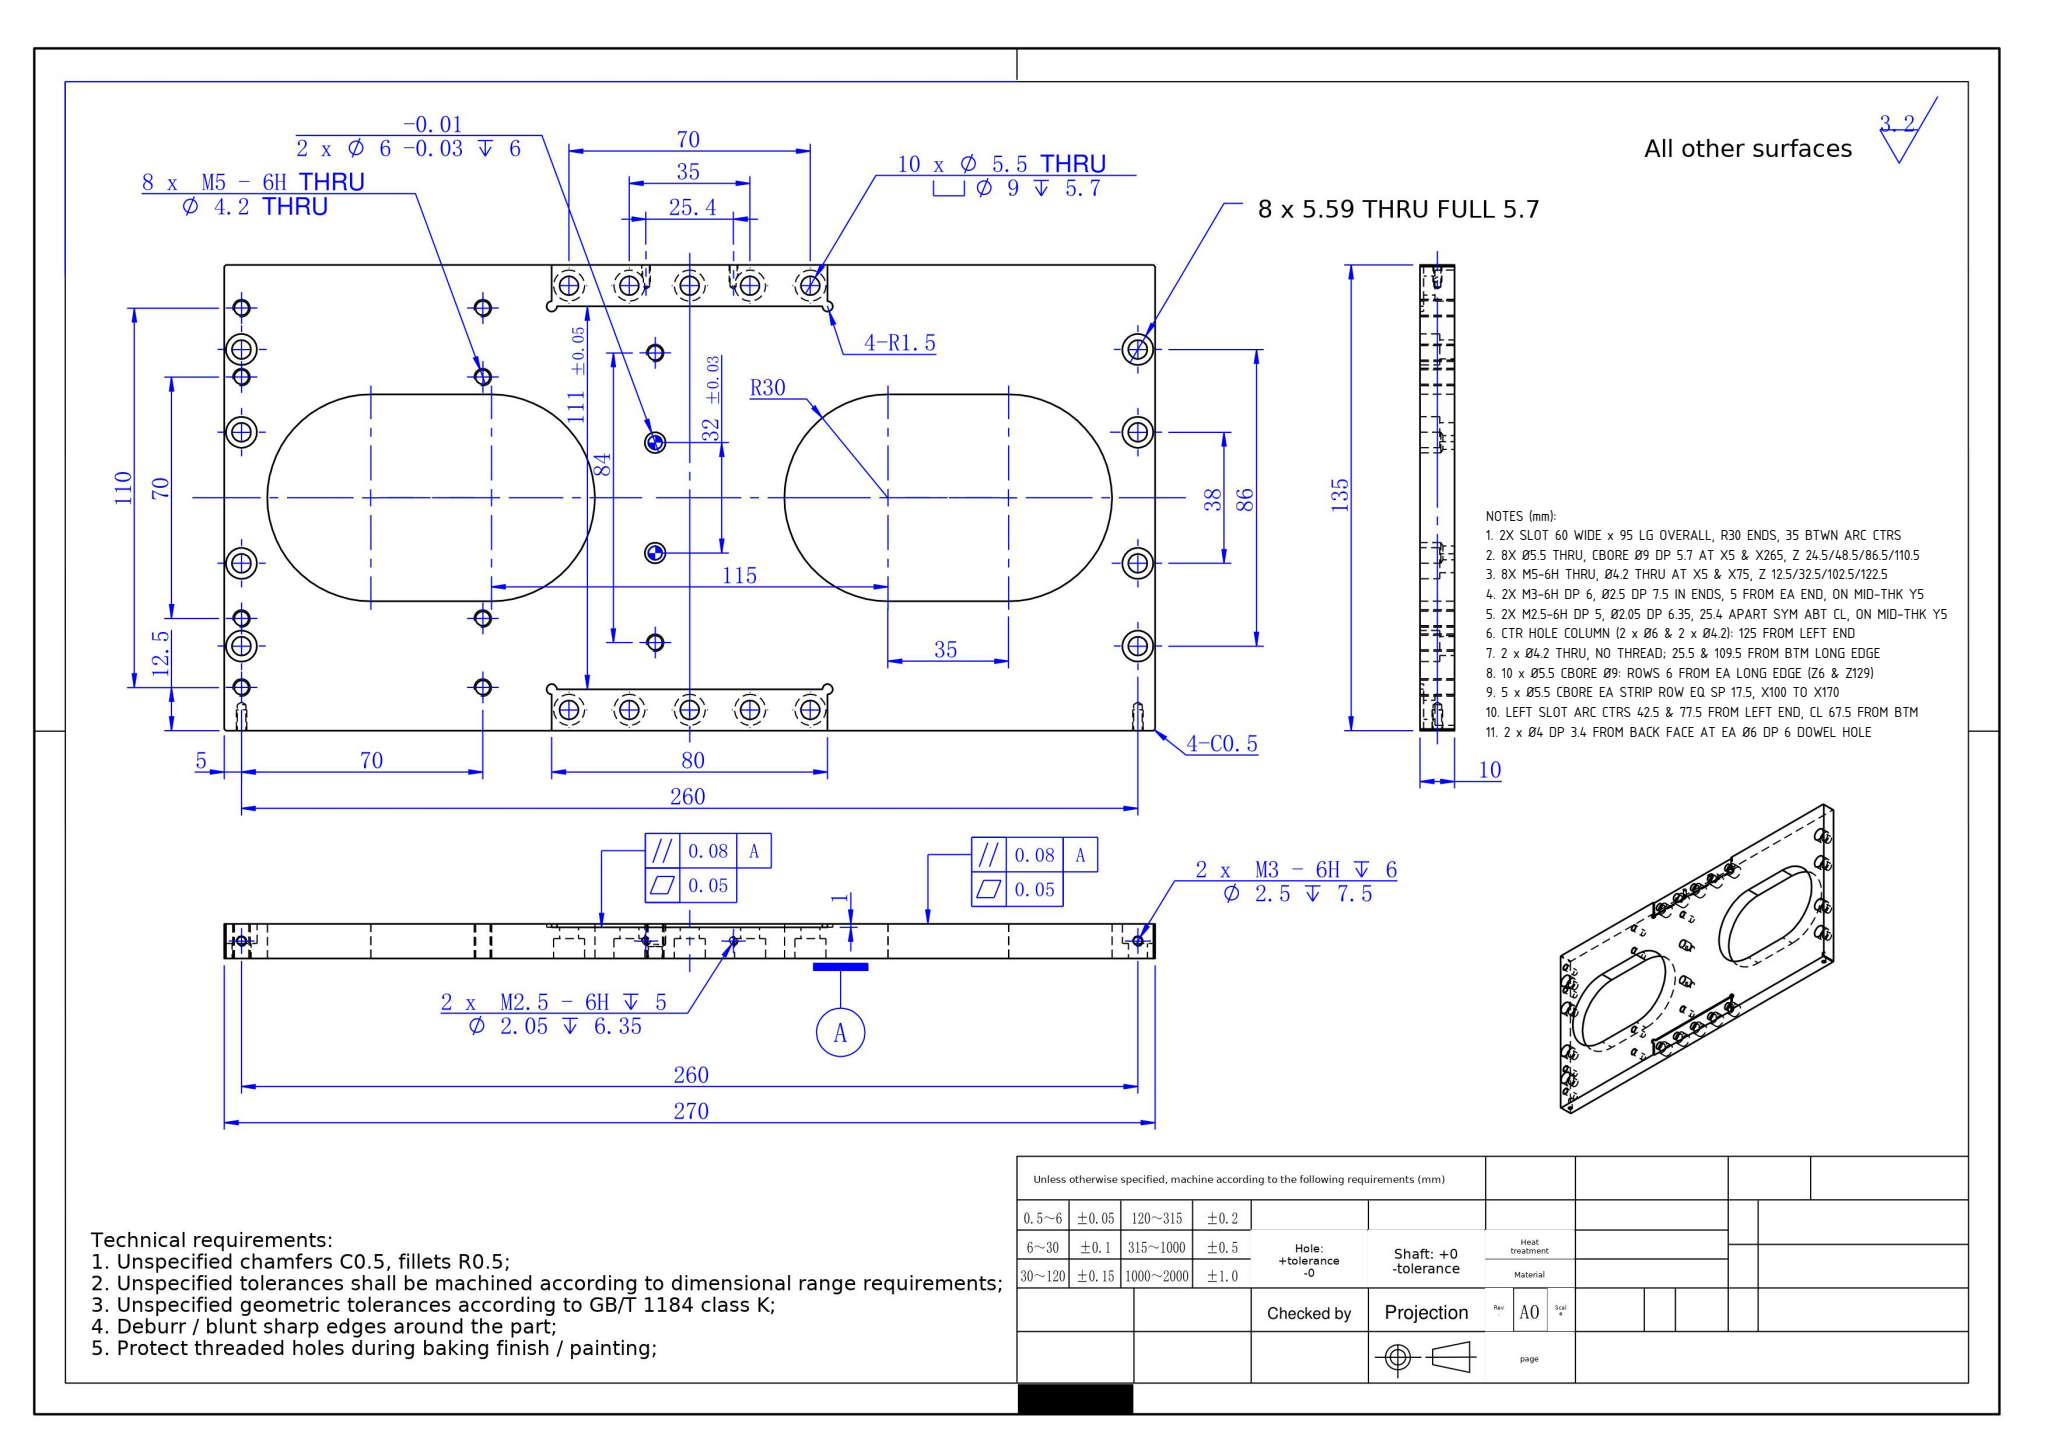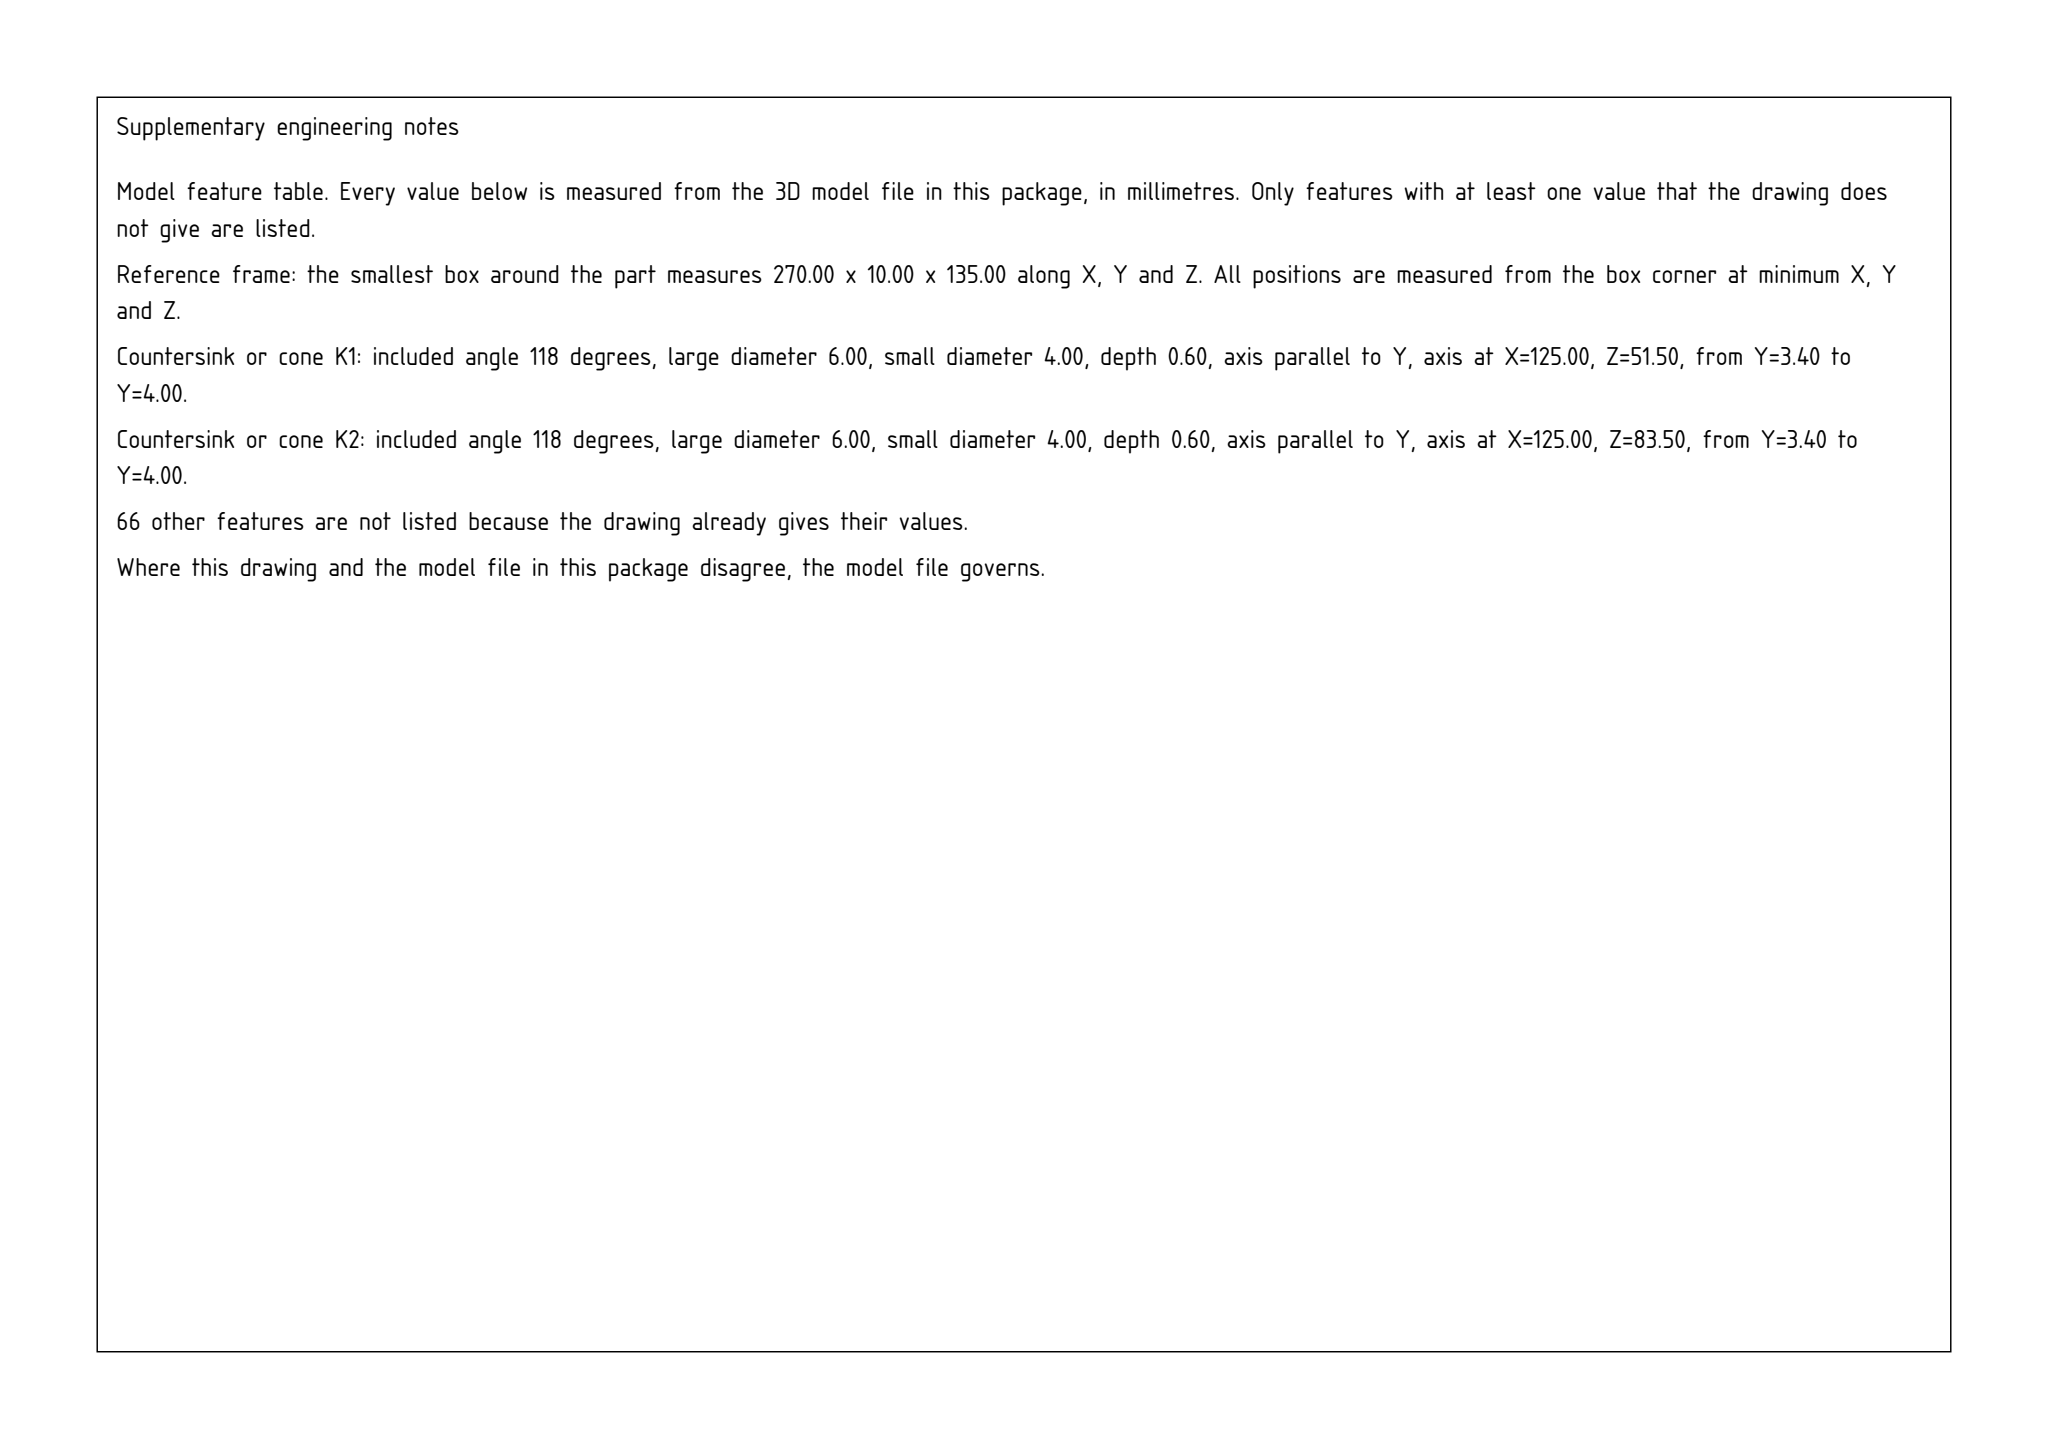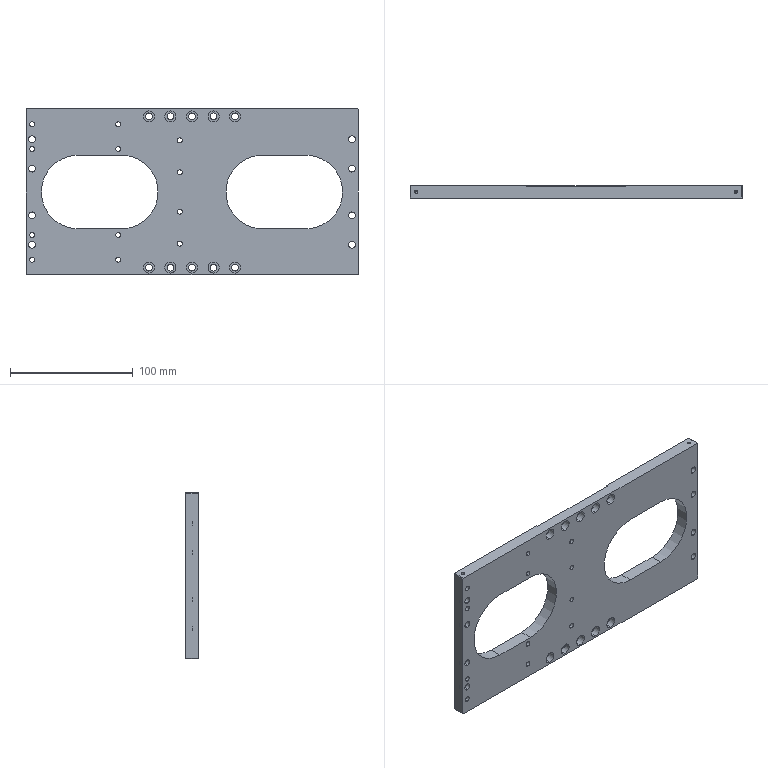Part | SolidWorks | mm | 1 solid | 170 faces | box 270 x 10 x 135 mm | volume 253927 mm3 | cylinder 118 | plane 40 | cone 12 | commonest cylinder face diameters 9 x36 5.5 x36 4.2 x20 3 x6 2.05 x4 6 x4 4 x4 2.5 x4
Drawing notes:
2X SLOT 60 WIDE x 95 LG OVERALL, R30 ENDS, 35 BTWN ARC CTRS | from the solid: Ø60 y-axis cyls at x=42.5 & 77.5 and x=192.5 & 227.5, z=67.5; 35 apart, 60+35=95
8X Ø5.5 THRU, CBORE Ø9 DP 5.7 AT X5 & X265, Z 24.5/48.5/86.5/110.5 | from the solid: Ø5.5 L4.3 + Ø9 L5.7 y-cyls at x=5 and x=265, z=24.5/48.5/86.5/110.5
8X M5-6H THRU, Ø4.2 THRU AT X5 & X75, Z 12.5/32.5/102.5/122.5 | from the solid: Ø4.2 y-axis thru holes at x=5 and x=75, z=12.5/32.5/102.5/122.5
2X M3-6H DP 6, Ø2.5 DP 7.5 IN ENDS, 5 FROM EA END, ON MID-THK Y5 | from the solid: Ø2.5 z-axis holes L7.5 at (x=5,y=5) and (x=265,y=5); bbox 270x10
2X M2.5-6H DP 5, Ø2.05 DP 6.35, 25.4 APART SYM ABT CL, ON MID-THK Y5 | from the solid: Ø2.05 z-axis holes L6.35 at x=122.3 & 147.7 (sym about x=135), y=5
CTR HOLE COLUMN (2 x Ø6 & 2 x Ø4.2): 125 FROM LEFT END | from the solid: Ø6 and Ø4.2 cylinders, axis Y, at x=125.0 (bbox X=270)
2 x Ø4.2 THRU, NO THREAD; 25.5 & 109.5 FROM BTM LONG EDGE | from the solid: Ø4.2 y-axis holes at [125,25.5] & [125,109.5], len 10 = full thk; no 4.2 thread cone
10 x Ø5.5 CBORE Ø9: ROWS 6 FROM EA LONG EDGE (Z6 & Z129) | from the solid: Ø5.5/Ø9 y-axis holes at z=6.0 and z=129.0 (bbox Z=135)
5 x Ø5.5 CBORE EA STRIP ROW EQ SP 17.5, X100 TO X170 | from the solid: x=100,117.5,135,152.5,170 for both z=6 and z=129 rows
LEFT SLOT ARC CTRS 42.5 & 77.5 FROM LEFT END, CL 67.5 FROM BTM | from the solid: Ø60 y-axis cyls at x=42.5 & 77.5 (and 192.5 & 227.5), z=67.5
2 x Ø4 DP 3.4 FROM BACK FACE AT EA Ø6 DP 6 DOWEL HOLE | from the solid: Ø4 y-axis cyls len 3.4 at [125,51.5] & [125,83.5], coaxial with Ø6 len 6
build123d program:
from build123d import *

# Parameters (mm, degrees)
SKETCH1_W                                            = 270
SKETCH1_H                                            = 135
BOSS_EXTRUDE1_DEPTH                                  = 5
CUT_EXTRUDE2_DEPTH                                   = 1
CHAMFER1_SIZE                                        = 0.5
M3_TAPPED_HOLE1_D                                    = 2.5
M3_TAPPED_HOLE1_DEPTH                                = 7.5
M3_TAPPED_HOLE1_TIP                                  = 0.7511
HOLE_SIZE_ACCORDING_TO_TYPE_OF_HEXAGON_S_D           = 5.5
HOLE_SIZE_ACCORDING_TO_TYPE_OF_HEXAGON_S_CBORE_D     = 9
HOLE_SIZE_ACCORDING_TO_TYPE_OF_HEXAGON_S_CBORE_DEPTH = 5.7
M5_TAPPED_HOLE2_D                                    = 4.2
HOLE_SIZE_ACCORDING_TO_TYPE_OF_HEXAG_2_D             = 5.5
HOLE_SIZE_ACCORDING_TO_TYPE_OF_HEXAG_2_CBORE_D       = 9
HOLE_SIZE_ACCORDING_TO_TYPE_OF_HEXAG_2_CBORE_DEPTH   = 5.7
M5_TAPPED_HOLE1_D                                    = 4.2
CUT_EXTRUDE4_DEPTH                                   = 152.265
F_4_0_4_DIAMETER_HOLE1_D                             = 4
SIZE_MM_DOWEL_PIN_HOLE2_D                            = 6
SIZE_MM_DOWEL_PIN_HOLE2_DEPTH                        = 6
SIZE_MM_DOWEL_PIN_HOLE2_TIP                          = 1.803
M2_5_TAPPED_HOLE1_D                                  = 2.05
M2_5_TAPPED_HOLE1_DEPTH                              = 6.35
M2_5_TAPPED_HOLE1_TIP                                = 0.6159


with BuildPart() as part:
    # Sketch1 → Boss-Extrude1 (new, symmetric)
    with BuildSketch(Plane(origin=(0, 0, 0), x_dir=(1, 0, 0), z_dir=(0, 1, 0))):
        Rectangle(SKETCH1_W, SKETCH1_H)
    extrude(amount=BOSS_EXTRUDE1_DEPTH, both=True)

    # Sketch2 → Cut-Extrude2 (cut)
    with BuildSketch(Plane(origin=(0, 5, 0), x_dir=(1, 0, 0), z_dir=(0, 1, 0))):
        with BuildLine():
            Line((0, -67.5), (0, -55.5))
            Line((0, -55.5), (-38.5, -55.5))
            ThreePointArc((-38.5, -55.5), (-38.939, -56.561), (-40, -57))
            Line((-40, -57), (-40, -67.5))
            Line((-40, -67.5), (0, -67.5))
        make_face()
        with BuildLine():
            Line((38.5, -55.5), (0, -55.5))
            Line((0, -55.5), (0, -67.5))
            Line((0, -67.5), (40, -67.5))
            Line((40, -67.5), (40, -57))
            ThreePointArc((40, -57), (38.939, -56.561), (38.5, -55.5))
        make_face()
        with BuildLine():
            ThreePointArc((41.5, -55.5), (40, -54), (38.5, -55.5))
            Line((38.5, -55.5), (40, -55.5))
            Line((40, -55.5), (40, -57))
            ThreePointArc((40, -57), (41.061, -56.561), (41.5, -55.5))
        make_face()
        with BuildLine():
            Line((40, -55.5), (38.5, -55.5))
            ThreePointArc((38.5, -55.5), (38.939, -56.561), (40, -57))
            Line((40, -57), (40, -55.5))
        make_face()
        with BuildLine():
            ThreePointArc((41.5, -55.5), (40, -54), (38.5, -55.5))
            Line((38.5, -55.5), (40, -55.5))
            Line((40, -55.5), (40, -57))
            ThreePointArc((40, -57), (41.061, -56.561), (41.5, -55.5))
        make_face()
        with BuildLine():
            Line((40, -55.5), (38.5, -55.5))
            ThreePointArc((38.5, -55.5), (38.939, -56.561), (40, -57))
            Line((40, -57), (40, -55.5))
        make_face()
        with BuildLine():
            ThreePointArc((-40, -57), (-38.939, -56.561), (-38.5, -55.5))
            Line((-38.5, -55.5), (-40, -55.5))
            Line((-40, -55.5), (-40, -57))
        make_face()
        with BuildLine():
            Line((-40, -55.5), (-38.5, -55.5))
            ThreePointArc((-38.5, -55.5), (-41.061, -54.439), (-40, -57))
            Line((-40, -57), (-40, -55.5))
        make_face()
        with BuildLine():
            ThreePointArc((-40, -57), (-38.939, -56.561), (-38.5, -55.5))
            Line((-38.5, -55.5), (-40, -55.5))
            Line((-40, -55.5), (-40, -57))
        make_face()
        with BuildLine():
            Line((-40, -55.5), (-38.5, -55.5))
            ThreePointArc((-38.5, -55.5), (-41.061, -54.439), (-40, -57))
            Line((-40, -57), (-40, -55.5))
        make_face()
    cut_extrude2 = extrude(amount=-CUT_EXTRUDE2_DEPTH, mode=Mode.SUBTRACT)

    # Mirror1: Cut-Extrude2 across plane
    add(cut_extrude2.mirror(Plane.XY), mode=Mode.SUBTRACT)

    # Chamfer1
    chamfer1_edges = [part.edges().sort_by_distance(p)[0] for p in [
        (135, 0, 67.5),
        (-135, 0, 67.5),
        (-135, 0, -67.5),
        (135, 0, -67.5),
    ]]
    chamfer(chamfer1_edges, length=CHAMFER1_SIZE)

    # M3 Tapped Hole1
    with Locations(Plane.XY.offset(67.5)):
        with Locations((-130, 0), (130, 0)):
            Hole(M3_TAPPED_HOLE1_D / 2, depth=M3_TAPPED_HOLE1_DEPTH)
            with Locations((0, 0, -(M3_TAPPED_HOLE1_DEPTH + M3_TAPPED_HOLE1_TIP / 2))):  # 118° drill point
                Cone(0, M3_TAPPED_HOLE1_D / 2, M3_TAPPED_HOLE1_TIP, mode=Mode.SUBTRACT)

    # Hole Size_According to_Type of Hexagon S (through all)
    with Locations(Plane(origin=(0, 5, 0), x_dir=(1, 0, 0), z_dir=(0, 1, 0))):
        with Locations((-130, 43), (-130, 19), (-130, -19), (-130, -43)):
            hole_size_according_to_type_of_hexagon_s = CounterBoreHole(HOLE_SIZE_ACCORDING_TO_TYPE_OF_HEXAGON_S_D / 2, HOLE_SIZE_ACCORDING_TO_TYPE_OF_HEXAGON_S_CBORE_D / 2, HOLE_SIZE_ACCORDING_TO_TYPE_OF_HEXAGON_S_CBORE_DEPTH)

    # Mirror7: Hole Size_According to_Type of Hexagon S across plane
    add(hole_size_according_to_type_of_hexagon_s.mirror(Plane(origin=(0, 0, 0), x_dir=(0, 0, 1), z_dir=(1, 0, 0))), mode=Mode.SUBTRACT)

    # M5 Tapped Hole2 (through all)
    with Locations(Plane(origin=(0, 5, 0), x_dir=(1, 0, 0), z_dir=(0, 1, 0))):
        with Locations((-130, -55), (-130, -35), (-130, 35), (-130, 55), (-60, -55), (-60, -35), (-60, 35), (-60, 55)):
            Hole(M5_TAPPED_HOLE2_D / 2)

    # Hole Size_According to_Type of Hexag 2 (through all)
    with Locations(Plane(origin=(0, -5, 0), x_dir=(-1, 0, 0), z_dir=(0, -1, 0))):
        with Locations((17.5, -61.5), (0, -61.5), (-17.5, -61.5), (-35, -61.5), (35, -61.5)):
            hole_size_according_to_type_of_hexag_2 = CounterBoreHole(HOLE_SIZE_ACCORDING_TO_TYPE_OF_HEXAG_2_D / 2, HOLE_SIZE_ACCORDING_TO_TYPE_OF_HEXAG_2_CBORE_D / 2, HOLE_SIZE_ACCORDING_TO_TYPE_OF_HEXAG_2_CBORE_DEPTH)

    # Mirror8: Hole Size_According to_Type of Hexag 2 across plane
    add(hole_size_according_to_type_of_hexag_2.mirror(Plane.XY), mode=Mode.SUBTRACT)

    # M5 Tapped Hole1 (through all)
    with Locations(Plane(origin=(0, 5, 0), x_dir=(1, 0, 0), z_dir=(0, 1, 0))):
        with Locations((-10, -42), (-10, 42)):
            Hole(M5_TAPPED_HOLE1_D / 2)

    # Sketch19 → Cut-Extrude4 (cut, through all)
    with BuildSketch(Plane(origin=(0, 5, 0), x_dir=(1, 0, 0), z_dir=(0, 1, 0))):
        with BuildLine():
            Line((-92.5, 30), (-57.5, 30))
            ThreePointArc((-57.5, 30), (-27.5, 0), (-57.5, -30))
            Line((-57.5, -30), (-92.5, -30))
            ThreePointArc((-92.5, -30), (-122.5, 0), (-92.5, 30))
        make_face()
        with BuildLine():
            Line((92.5, 30), (57.5, 30))
            ThreePointArc((57.5, 30), (27.5, 0), (57.5, -30))
            Line((57.5, -30), (92.5, -30))
            ThreePointArc((92.5, -30), (122.5, 0), (92.5, 30))
        make_face()
    extrude(amount=-CUT_EXTRUDE4_DEPTH, mode=Mode.SUBTRACT)

    # 4.0 _4_ Diameter Hole1 (through all)
    with Locations(Plane(origin=(0, -5, 0), x_dir=(-1, 0, 0), z_dir=(0, -1, 0))):
        with Locations((10, 16), (10, -16)):
            Hole(F_4_0_4_DIAMETER_HOLE1_D / 2)

    # Size mm Dowel Pin Hole2
    with Locations(Plane(origin=(0, 5, 0), x_dir=(1, 0, 0), z_dir=(0, 1, 0))):
        with Locations((-10, 16), (-10, -16)):
            Hole(SIZE_MM_DOWEL_PIN_HOLE2_D / 2, depth=SIZE_MM_DOWEL_PIN_HOLE2_DEPTH)
            with Locations((0, 0, -(SIZE_MM_DOWEL_PIN_HOLE2_DEPTH + SIZE_MM_DOWEL_PIN_HOLE2_TIP / 2))):  # 118° drill point
                Cone(0, SIZE_MM_DOWEL_PIN_HOLE2_D / 2, SIZE_MM_DOWEL_PIN_HOLE2_TIP, mode=Mode.SUBTRACT)

    # M2.5 Tapped Hole1
    with Locations(Plane(origin=(0, 0, -67.5), x_dir=(-1, 0, 0), z_dir=(0, 0, -1))):
        with Locations((-12.7, 0), (12.7, 0)):
            Hole(M2_5_TAPPED_HOLE1_D / 2, depth=M2_5_TAPPED_HOLE1_DEPTH)
            with Locations((0, 0, -(M2_5_TAPPED_HOLE1_DEPTH + M2_5_TAPPED_HOLE1_TIP / 2))):  # 118° drill point
                Cone(0, M2_5_TAPPED_HOLE1_D / 2, M2_5_TAPPED_HOLE1_TIP, mode=Mode.SUBTRACT)


solid = part.part